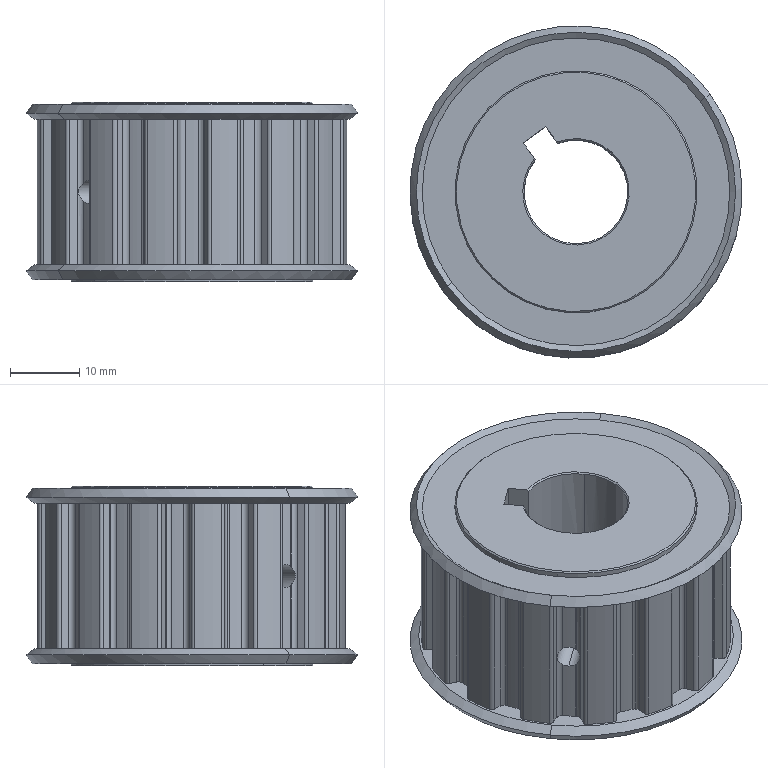Component | SolidWorks | ATPA15L075_A_H15-01-2-1 | 1 solid | 179 faces | box 48 x 48 x 26 mm | volume 32681 mm3 | cylinder 121 | plane 41 | cone 17 | commonest cylinder face diameters 1.06 x37 1.72 x37 40.46 x17 44.72 x15 3.3 x8 35 x4 15 x3
build123d program:
from build123d import *

# Parameters (mm, degrees)
SKETCH2_W              = 12
SKETCH2_H              = 17.5
SKETCH3_W              = 89.44
SKETCH3_H              = 89.44
CUT_EXTRUDE1_DEPTH     = 21
SKETCH4_W              = 4
SKETCH4_H              = 3
CUT_EXTRUDE2_DEPTH     = 43.755
M4_TAPPED_HOLE1_REACH  = 55.052
M4_TAPPED_HOLE1_BORE_R = 1.65
M4_TAPPED_HOLE2_D      = 3.3
M4_TAPPED_HOLE2_DEPTH  = 46.607
M4_TAPPED_HOLE2_TIP    = 0.9914


with BuildPart() as part:
    # Sketch1 → Revolve1 (revolve)
    with BuildSketch(Plane.XY, mode=Mode.PRIVATE) as revolve1_sk:
        Polygon((0, 17.3), (0, 7.7), (0.2, 7.5), (37.8, 7.5), (38, 7.7), (38, 8.3), (37.8, 8.5), (26, 8.5), (26, 17.5), (25.1, 17.5), (25.1, 22.227), (25.702, 23.07), (24.4, 24), (23.5, 22.74), (2.5, 22.74), (1.6, 24), (0.298, 23.07), (0.9, 22.227), (0.9, 17.5), (0.2, 17.5), align=None)
    revolve(revolve1_sk.sketch.rotate(Axis((38, 0, 0), (-1, 0, 0)), 270), axis=Axis((38, 0, 0), (-1, 0, 0)))

    # Sketch2 → Cut-Revolve1 (revolve, cut)
    with BuildSketch(Plane.XY, mode=Mode.PRIVATE) as cut_revolve1_sk:
        with Locations((32, 8.75)):
            Rectangle(SKETCH2_W, SKETCH2_H)
    revolve(cut_revolve1_sk.sketch.rotate(Axis((38, 0, 0), (-1, 0, 0)), 270), axis=Axis((38, 0, 0), (-1, 0, 0)), mode=Mode.SUBTRACT)

    # Sketch3 → Cut-Extrude1 (cut)
    with BuildSketch(Plane(origin=(2.5, 0, 0), x_dir=(0, 0, -1), z_dir=(1, 0, 0))):
        Rectangle(SKETCH3_W, SKETCH3_H)
        with BuildLine():
            Line((-21.955, -0.1348), (-20.845, -0.4115))
            ThreePointArc((-20.845, -0.4115), (-20.391, -0.6967), (-20.195, -1.195))
            ThreePointArc((-20.195, -1.195), (-20.119, -2.115), (-20.002, -3.03))
            ThreePointArc((-20.002, -3.03), (-20.091, -3.558), (-20.475, -3.931))
            Line((-20.475, -3.931), (-21.503, -4.433))
            ThreePointArc((-21.503, -4.433), (-21.749, -4.681), (-21.787, -5.028))
            ThreePointArc((-21.787, -5.028), (-21.547, -5.975), (-21.266, -6.91))
            ThreePointArc((-21.266, -6.91), (-20.944, -7.831), (-20.582, -8.738))
            ThreePointArc((-20.582, -8.738), (-20.347, -8.997), (-20.002, -9.053))
            Line((-20.002, -9.053), (-18.876, -8.854))
            ThreePointArc((-18.876, -8.854), (-18.345, -8.93), (-17.963, -9.306))
            ThreePointArc((-17.963, -9.306), (-17.52, -10.115), (-17.04, -10.903))
            ThreePointArc((-17.04, -10.903), (-16.907, -11.422), (-17.106, -11.92))
            Line((-17.106, -11.92), (-17.841, -12.796))
            ThreePointArc((-17.841, -12.796), (-17.965, -13.122), (-17.858, -13.455))
            ThreePointArc((-17.858, -13.455), (-17.254, -14.222), (-16.617, -14.962))
            ThreePointArc((-16.617, -14.962), (-15.948, -15.673), (-15.248, -16.354))
            ThreePointArc((-15.248, -16.354), (-14.928, -16.495), (-14.591, -16.406))
            Line((-14.591, -16.406), (-13.642, -15.766))
            ThreePointArc((-13.642, -15.766), (-13.127, -15.62), (-12.625, -15.807))
            ThreePointArc((-12.625, -15.807), (-11.891, -16.366), (-11.132, -16.891))
            ThreePointArc((-11.132, -16.891), (-10.799, -17.311), (-10.779, -17.847))
            Line((-10.779, -17.847), (-11.094, -18.946))
            ThreePointArc((-11.094, -18.946), (-11.074, -19.295), (-10.842, -19.556))
            ThreePointArc((-10.842, -19.556), (-9.978, -20.01), (-9.095, -20.427))
            ThreePointArc((-9.095, -20.427), (-8.194, -20.804), (-7.278, -21.142))
            ThreePointArc((-7.278, -21.142), (-6.929, -21.141), (-6.656, -20.922))
            Line((-6.656, -20.922), (-6.05, -19.952))
            ThreePointArc((-6.05, -19.952), (-5.639, -19.609), (-5.104, -19.576))
            ThreePointArc((-5.104, -19.576), (-4.206, -19.788), (-3.3, -19.959))
            ThreePointArc((-3.3, -19.959), (-2.824, -20.207), (-2.588, -20.688))
            Line((-2.588, -20.688), (-2.429, -21.821))
            ThreePointArc((-2.429, -21.821), (-2.269, -22.131), (-1.95, -22.275))
            ThreePointArc((-1.95, -22.275), (-0.9761, -22.339), (0, -22.36))
            ThreePointArc((0, -22.36), (0.9761, -22.339), (1.95, -22.275))
            ThreePointArc((1.95, -22.275), (2.269, -22.131), (2.429, -21.821))
            Line((2.429, -21.821), (2.588, -20.688))
            ThreePointArc((2.588, -20.688), (2.824, -20.207), (3.3, -19.959))
            ThreePointArc((3.3, -19.959), (4.206, -19.788), (5.104, -19.576))
            ThreePointArc((5.104, -19.576), (5.639, -19.609), (6.05, -19.952))
            Line((6.05, -19.952), (6.656, -20.922))
            ThreePointArc((6.656, -20.922), (6.929, -21.141), (7.278, -21.142))
            ThreePointArc((7.278, -21.142), (8.194, -20.804), (9.095, -20.427))
            ThreePointArc((9.095, -20.427), (9.978, -20.01), (10.842, -19.556))
            ThreePointArc((10.842, -19.556), (11.074, -19.295), (11.094, -18.946))
            Line((11.094, -18.946), (10.779, -17.847))
            ThreePointArc((10.779, -17.847), (10.799, -17.311), (11.132, -16.891))
            ThreePointArc((11.132, -16.891), (11.891, -16.366), (12.625, -15.807))
            ThreePointArc((12.625, -15.807), (13.127, -15.62), (13.642, -15.766))
            Line((13.642, -15.766), (14.591, -16.406))
            ThreePointArc((14.591, -16.406), (14.928, -16.495), (15.248, -16.354))
            ThreePointArc((15.248, -16.354), (15.948, -15.673), (16.617, -14.962))
            ThreePointArc((16.617, -14.962), (17.254, -14.222), (17.858, -13.455))
            ThreePointArc((17.858, -13.455), (17.965, -13.122), (17.841, -12.796))
            Line((17.841, -12.796), (17.106, -11.92))
            ThreePointArc((17.106, -11.92), (16.907, -11.422), (17.04, -10.903))
            ThreePointArc((17.04, -10.903), (17.52, -10.115), (17.963, -9.306))
            ThreePointArc((17.963, -9.306), (18.345, -8.93), (18.876, -8.854))
            Line((18.876, -8.854), (20.002, -9.053))
            ThreePointArc((20.002, -9.053), (20.347, -8.997), (20.582, -8.738))
            ThreePointArc((20.582, -8.738), (20.944, -7.831), (21.266, -6.91))
            ThreePointArc((21.266, -6.91), (21.547, -5.975), (21.787, -5.028))
            ThreePointArc((21.787, -5.028), (21.749, -4.681), (21.503, -4.433))
            Line((21.503, -4.433), (20.475, -3.931))
            ThreePointArc((20.475, -3.931), (20.091, -3.558), (20.002, -3.03))
            ThreePointArc((20.002, -3.03), (20.119, -2.115), (20.195, -1.195))
            ThreePointArc((20.195, -1.195), (20.391, -0.6967), (20.845, -0.4115))
            Line((20.845, -0.4115), (21.955, -0.1348))
            ThreePointArc((21.955, -0.1348), (22.247, 0.05676), (22.357, 0.3886))
            ThreePointArc((22.357, 0.3886), (22.318, 1.364), (22.238, 2.337))
            ThreePointArc((22.238, 2.337), (22.114, 3.306), (21.949, 4.268))
            ThreePointArc((21.949, 4.268), (21.773, 4.57), (21.447, 4.697))
            Line((21.447, 4.697), (20.304, 4.736))
            ThreePointArc((20.304, 4.736), (19.801, 4.921), (19.505, 5.368))
            ThreePointArc((19.505, 5.368), (19.24, 6.251), (18.935, 7.122))
            ThreePointArc((18.935, 7.122), (18.912, 7.657), (19.21, 8.103))
            Line((19.21, 8.103), (20.112, 8.807))
            ThreePointArc((20.112, 8.807), (20.301, 9.101), (20.266, 9.448))
            ThreePointArc((20.266, 9.448), (19.834, 10.324), (19.364, 11.18))
            ThreePointArc((19.364, 11.18), (18.858, 12.015), (18.315, 12.826))
            ThreePointArc((18.315, 12.826), (18.032, 13.031), (17.683, 13.014))
            Line((17.683, 13.014), (16.622, 12.585))
            ThreePointArc((16.622, 12.585), (16.087, 12.549), (15.635, 12.837))
            ThreePointArc((15.635, 12.837), (15.034, 13.537), (14.401, 14.208))
            ThreePointArc((14.401, 14.208), (14.162, 14.688), (14.254, 15.216))
            Line((14.254, 15.216), (14.791, 16.225))
            ThreePointArc((14.791, 16.225), (14.844, 16.571), (14.671, 16.874))
            ThreePointArc((14.671, 16.874), (13.92, 17.499), (13.143, 18.09))
            ThreePointArc((13.143, 18.09), (12.341, 18.646), (11.515, 19.167))
            ThreePointArc((11.515, 19.167), (11.173, 19.238), (10.861, 19.081))
            Line((10.861, 19.081), (10.066, 18.258))
            ThreePointArc((10.066, 18.258), (9.592, 18.008), (9.062, 18.087))
            ThreePointArc((9.062, 18.087), (8.228, 18.481), (7.377, 18.837))
            ThreePointArc((7.377, 18.837), (6.964, 19.178), (6.833, 19.698))
            Line((6.833, 19.698), (6.913, 20.839))
            ThreePointArc((6.913, 20.839), (6.821, 21.176), (6.539, 21.383))
            ThreePointArc((6.539, 21.383), (5.599, 21.648), (4.649, 21.871))
            ThreePointArc((4.649, 21.871), (3.69, 22.053), (2.723, 22.194))
            ThreePointArc((2.723, 22.194), (2.382, 22.119), (2.161, 21.849))
            Line((2.161, 21.849), (1.77, 20.774))
            ThreePointArc((1.77, 20.774), (1.439, 20.353), (0.9223, 20.209))
            ThreePointArc((0.9223, 20.209), (0, 20.23), (-0.9223, 20.209))
            ThreePointArc((-0.9223, 20.209), (-1.439, 20.353), (-1.77, 20.774))
            Line((-1.77, 20.774), (-2.161, 21.849))
            ThreePointArc((-2.161, 21.849), (-2.382, 22.119), (-2.723, 22.194))
            ThreePointArc((-2.723, 22.194), (-3.69, 22.053), (-4.649, 21.871))
            ThreePointArc((-4.649, 21.871), (-5.599, 21.648), (-6.539, 21.383))
            ThreePointArc((-6.539, 21.383), (-6.821, 21.176), (-6.913, 20.839))
            Line((-6.913, 20.839), (-6.833, 19.698))
            ThreePointArc((-6.833, 19.698), (-6.964, 19.178), (-7.377, 18.837))
            ThreePointArc((-7.377, 18.837), (-8.228, 18.481), (-9.062, 18.087))
            ThreePointArc((-9.062, 18.087), (-9.592, 18.008), (-10.066, 18.258))
            Line((-10.066, 18.258), (-10.861, 19.081))
            ThreePointArc((-10.861, 19.081), (-11.173, 19.238), (-11.515, 19.167))
            ThreePointArc((-11.515, 19.167), (-12.341, 18.646), (-13.143, 18.09))
            ThreePointArc((-13.143, 18.09), (-13.92, 17.499), (-14.671, 16.874))
            ThreePointArc((-14.671, 16.874), (-14.844, 16.571), (-14.791, 16.225))
            Line((-14.791, 16.225), (-14.254, 15.216))
            ThreePointArc((-14.254, 15.216), (-14.162, 14.688), (-14.401, 14.208))
            ThreePointArc((-14.401, 14.208), (-15.034, 13.537), (-15.635, 12.837))
            ThreePointArc((-15.635, 12.837), (-16.087, 12.549), (-16.622, 12.585))
            Line((-16.622, 12.585), (-17.683, 13.014))
            ThreePointArc((-17.683, 13.014), (-18.032, 13.031), (-18.315, 12.826))
            ThreePointArc((-18.315, 12.826), (-18.858, 12.015), (-19.364, 11.18))
            ThreePointArc((-19.364, 11.18), (-19.834, 10.324), (-20.266, 9.448))
            ThreePointArc((-20.266, 9.448), (-20.301, 9.101), (-20.112, 8.807))
            Line((-20.112, 8.807), (-19.21, 8.103))
            ThreePointArc((-19.21, 8.103), (-18.912, 7.657), (-18.935, 7.122))
            ThreePointArc((-18.935, 7.122), (-19.24, 6.251), (-19.505, 5.368))
            ThreePointArc((-19.505, 5.368), (-19.801, 4.921), (-20.304, 4.736))
            Line((-20.304, 4.736), (-21.447, 4.697))
            ThreePointArc((-21.447, 4.697), (-21.773, 4.57), (-21.949, 4.268))
            ThreePointArc((-21.949, 4.268), (-22.114, 3.306), (-22.238, 2.337))
            ThreePointArc((-22.238, 2.337), (-22.318, 1.364), (-22.357, 0.3886))
            ThreePointArc((-22.357, 0.3886), (-22.247, 0.05676), (-21.955, -0.1348))
        make_face(mode=Mode.SUBTRACT)
    extrude(amount=CUT_EXTRUDE1_DEPTH, mode=Mode.SUBTRACT)

    # Sketch4 → Cut-Extrude2 (cut, through all)
    with BuildSketch(Plane(origin=(26, 0, 0), x_dir=(0, 0, -1), z_dir=(1, 0, 0))):
        with Locations((0, 8.728)):
            Rectangle(SKETCH4_W, SKETCH4_H)
    extrude(amount=-CUT_EXTRUDE2_DEPTH, mode=Mode.SUBTRACT)

    # M4 Tapped Hole1 bore (on position points) → M4 Tapped Hole1 (cut, up to next)
    with BuildSketch(Plane(origin=(12.36, -2.115, 20.119), x_dir=(0, 0.9945, 0.1045), z_dir=(0, -0.1045, 0.9945)), mode=Mode.PRIVATE) as m4_tapped_hole1_sk1:
        Circle(M4_TAPPED_HOLE1_BORE_R)
    m4_tapped_hole1_tool1 = extrude(m4_tapped_hole1_sk1.sketch, amount=-M4_TAPPED_HOLE1_REACH, mode=Mode.PRIVATE) & part.part
    add(m4_tapped_hole1_tool1.solids().sort_by_distance((12.36, -2.115, 20.119))[0], mode=Mode.SUBTRACT)

    # M4 Tapped Hole2
    with Locations(Plane(origin=(0, 0, -23), x_dir=(1, 0, 0), z_dir=(0, 0, -1))):
        with Locations((13, 2.112)):
            Hole(M4_TAPPED_HOLE2_D / 2, depth=M4_TAPPED_HOLE2_DEPTH)
            with Locations((0, 0, -(M4_TAPPED_HOLE2_DEPTH + M4_TAPPED_HOLE2_TIP / 2))):  # 118° drill point
                Cone(0, M4_TAPPED_HOLE2_D / 2, M4_TAPPED_HOLE2_TIP, mode=Mode.SUBTRACT)


solid = part.part

# Placed as in the assembly
solid = solid.moved(Location((499.783, -234.615, -173), (-90, 53.906, 90)))